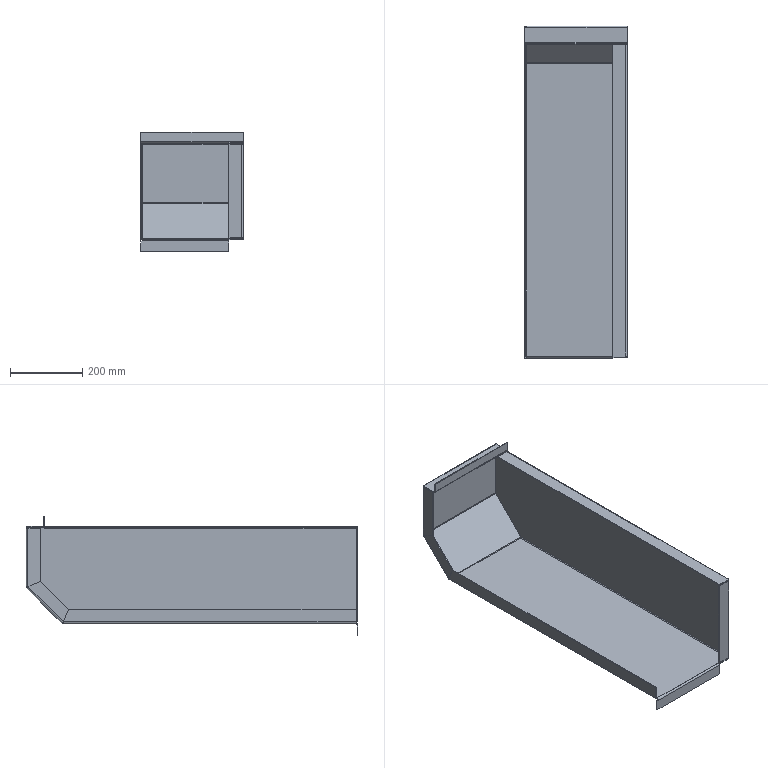Component | NX | SIDE_COLUMN_REAR_RIGHT | 1 solid | 93 faces | volume 1337463 mm3 | plane 70 | cylinder 23 | commonest cylinder face diameters 6 x12 10 x11